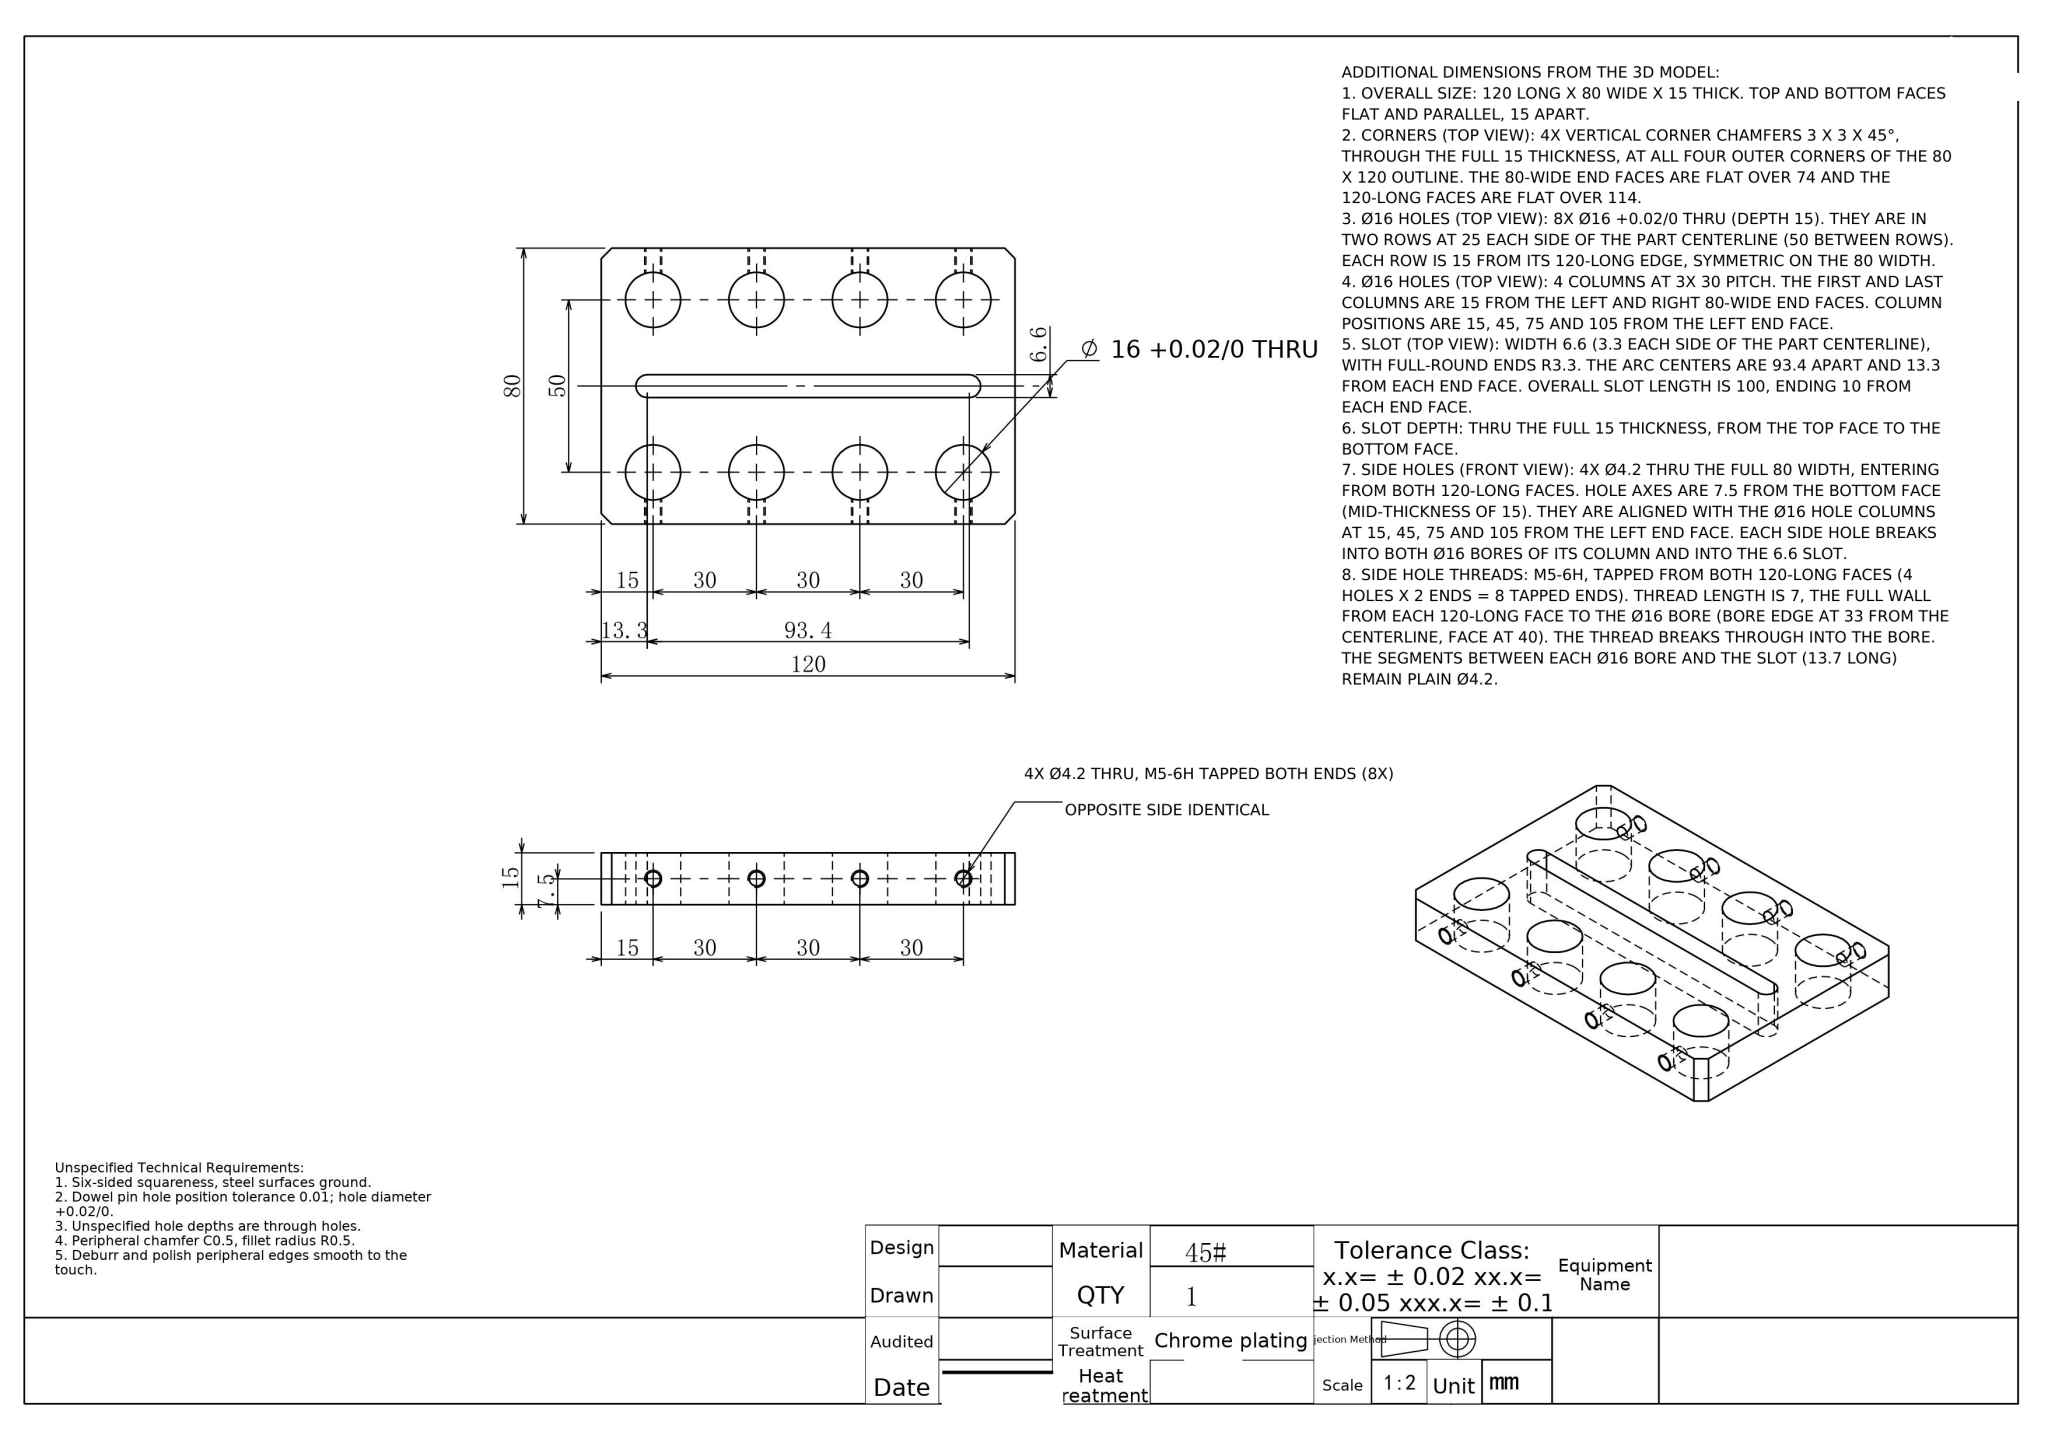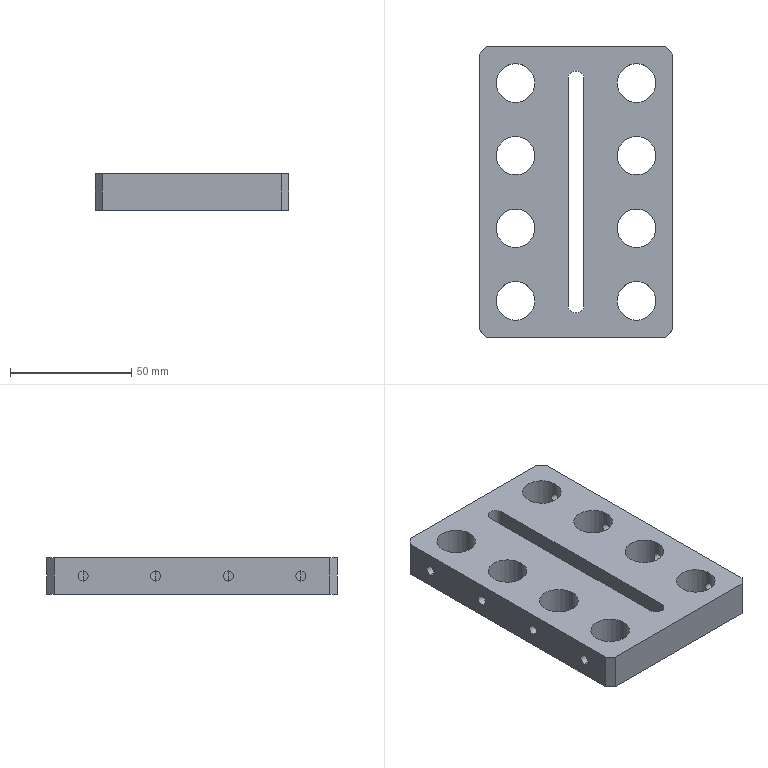Part | NX | mm | 1 solid | 46 faces | box 80 x 120 x 15 mm | volume 109059 mm3 | cylinder 34 | plane 12 | commonest cylinder face diameters 4.2 x16 16 x16 6.6 x2